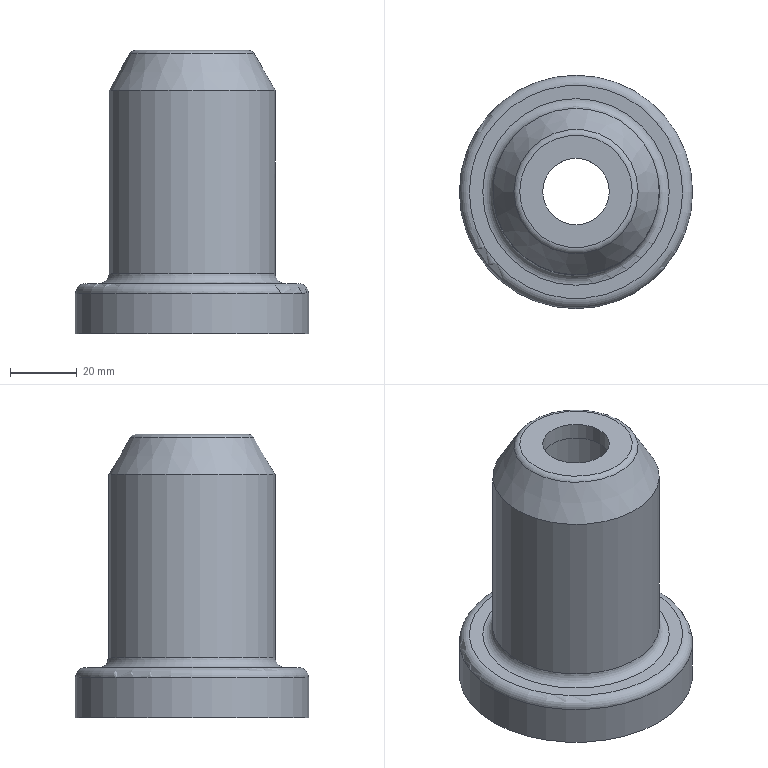Component | NX | AIR_CYLINDER | 1 solid | 36 faces | volume 103215 mm3 | cylinder 13 | cone 13 | plane 6 | torus 4 | commonest cylinder face diameters 6 x6 50 x1 28 x1 70 x1 46 x1 40 x1 20 x1 3 x1